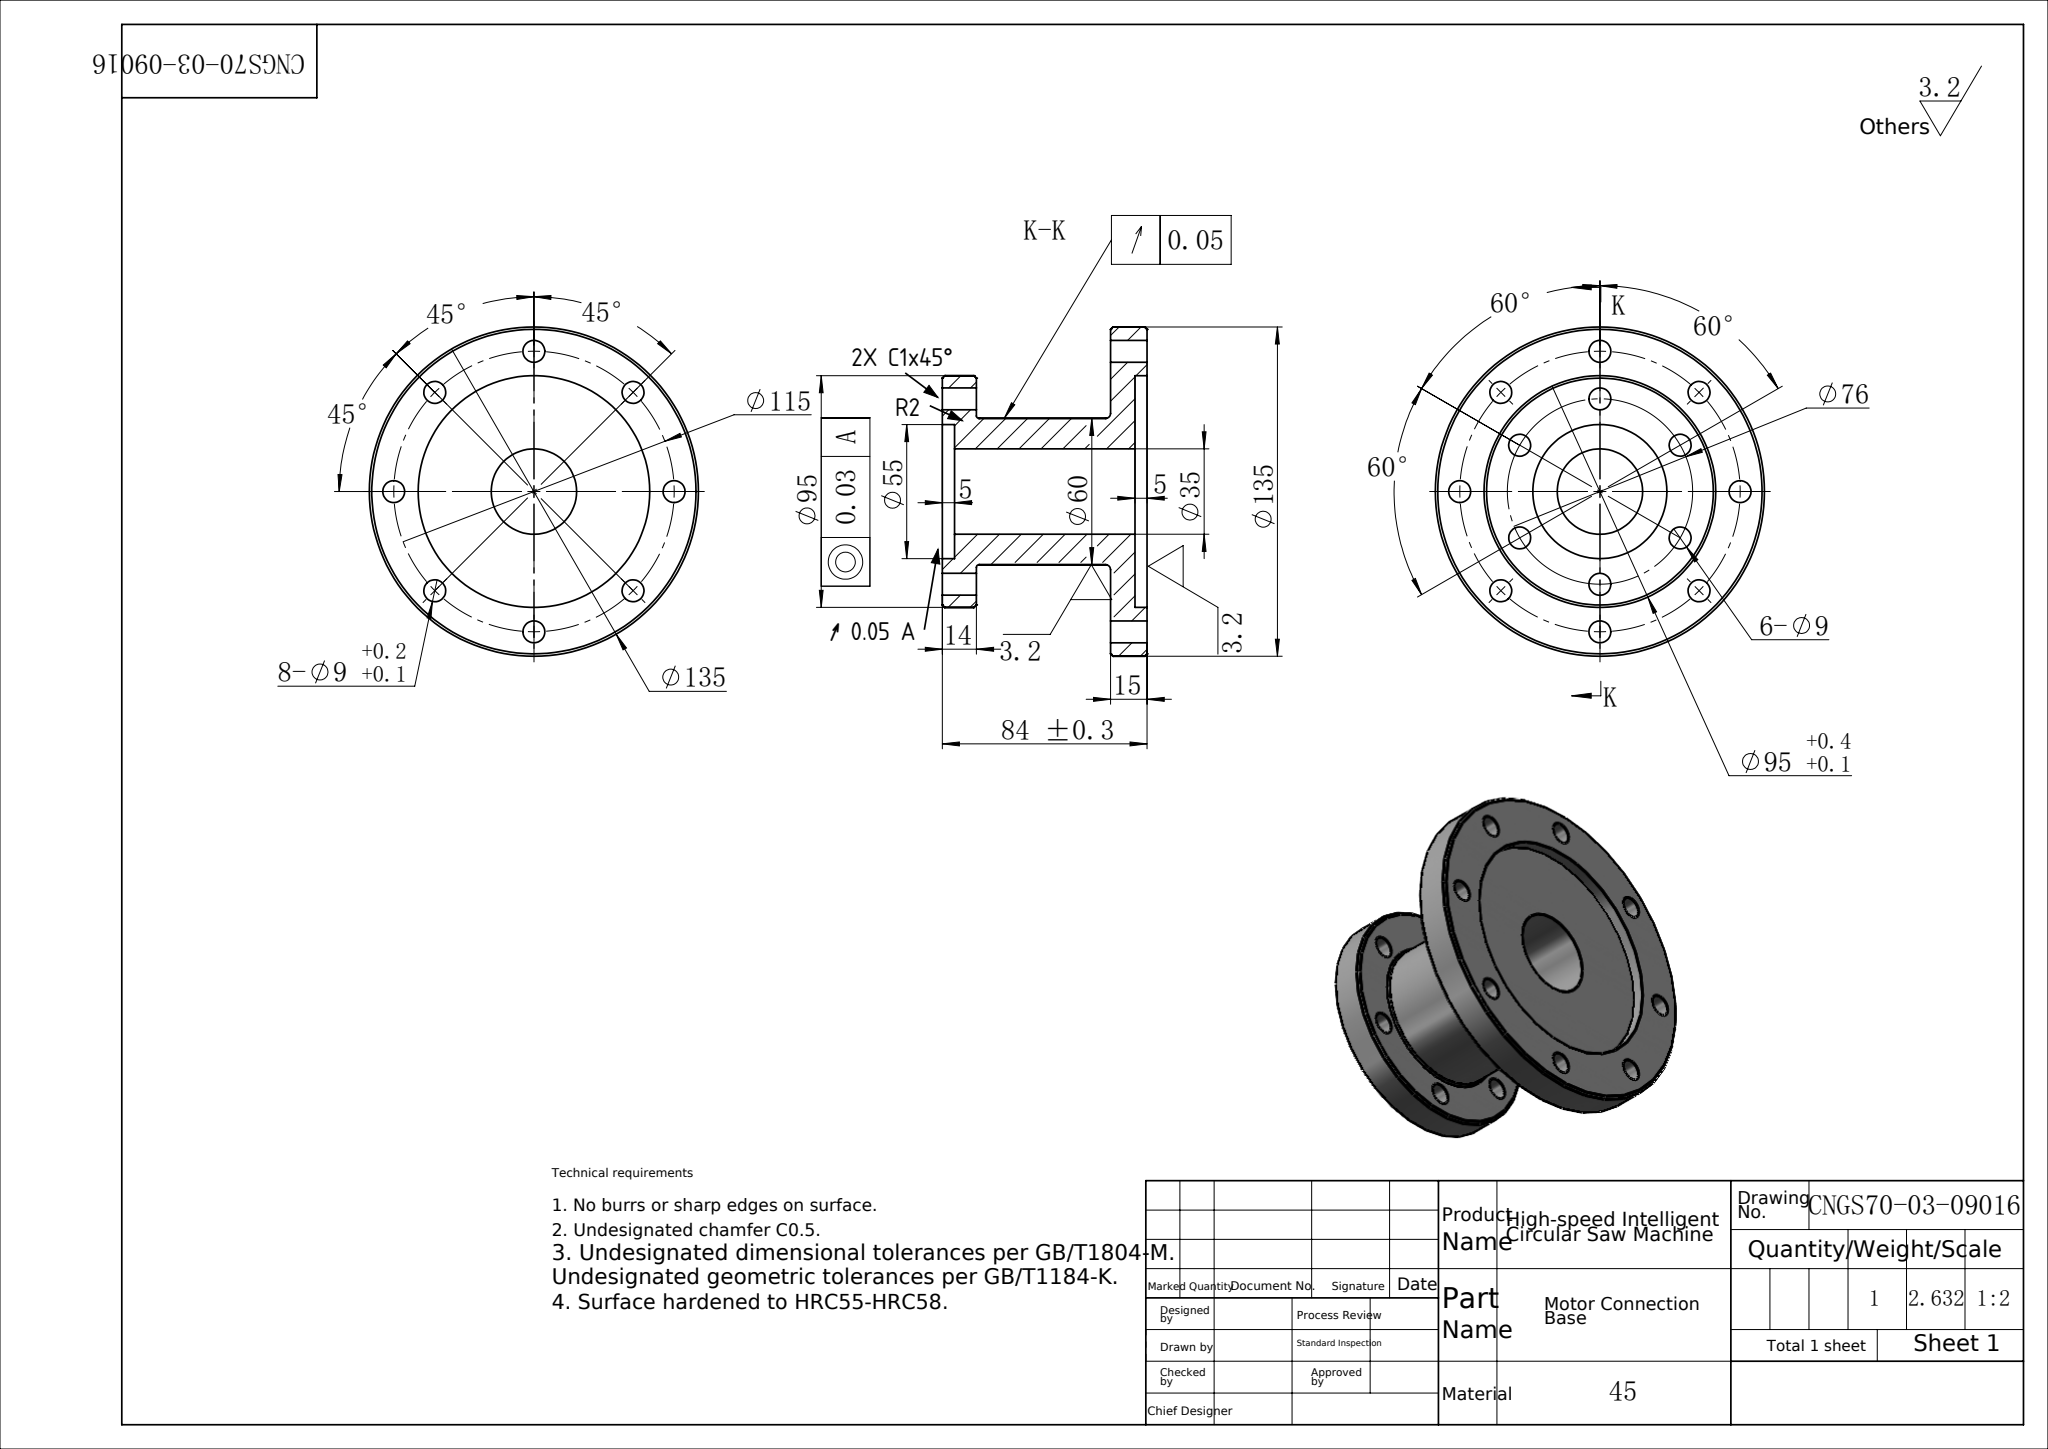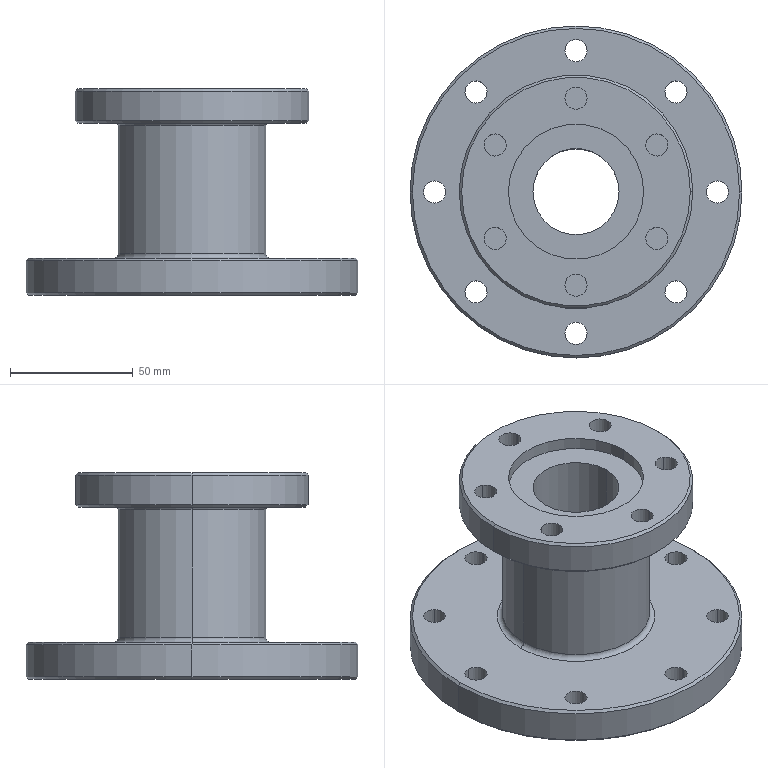Part | SolidWorks | mm | material 45 | 1 solid | 58 faces | box 135 x 135 x 84 mm | volume 337444 mm3 | cylinder 40 | cone 8 | plane 6 | torus 4 | commonest cylinder face diameters 9 x28 95 x4 55 x2 135 x2 60 x2 35 x2
Drawing notes:
K-K: CIRCULAR RUNOUT ↗ 0.05 OF Ø95 FLANGE FACE TO DATUM A | from the solid: Ø95 cyl, axis z at (67.5,67.5), faces at z=0/5 and z=79/84 coaxial with Ø60 hub (L=52) and Ø35 bore (L=74); flange faces are planes normal to z at 0,5,79,84
UNNOTED FILLETS R2 AT HUB-TO-FLANGE TRANSITIONS, R1 ALL OTHERS | from the solid: fillet_radii: [[2.0, 2], [1.0, 2]] - two R2 and two R1 blends on hub/flange junctions in section K-K
C1 x 45° BOTH EDGES OF Ø95 FLANGE (SEE K-K) | from the solid: cones 90° incl, ref dia 95 & 93 (2 ea) at Ø95 flange faces = 1 mm x 45° chamfer
build123d program:
from build123d import *

# Parameters (mm, degrees)
SKETCH1_R                     = 47.5
BOSS_EXTRUDE1_DEPTH           = 14
SIZE_MM_DOWEL_PIN_HOLE1_D     = 9
SIZE_MM_DOWEL_PIN_HOLE1_DEPTH = 14
SKETCH5_R                     = 30
BOSS_EXTRUDE2_DEPTH           = 55
SKETCH6_R                     = 67.5
BOSS_EXTRUDE3_DEPTH           = 15
SKETCH7_R                     = 47.5
CUT_EXTRUDE3_DEPTH            = 5
FILLET1_R                     = 1
FILLET2_R                     = 2
CHAMFER1_SIZE                 = 1
SKETCH10_R                    = 17.5
CUT_EXTRUDE4_DEPTH            = 124.909
SKETCH2_R                     = 31
SKETCH2_R_2                   = 25
BOSS_EXTRUDE4_DEPTH           = 3.5
CUT_EXTRUDE5_START            = -3.5
SKETCH11_R                    = 31
CUT_EXTRUDE5_DEPTH            = 3.5
SKETCH12_R                    = 27.5
CUT_EXTRUDE6_DEPTH            = 5
CIRPATTERN1_COUNT             = 8
CIRPATTERN2_COUNT             = 6


with BuildPart() as part:
    # Sketch1 → Boss-Extrude1 (new body)
    with BuildSketch(Plane.XY):
        Circle(SKETCH1_R)
    extrude(amount=BOSS_EXTRUDE1_DEPTH)

    # Size mm Dowel Pin Hole1
    with Locations(Plane(origin=(0, 0, 0), x_dir=(-1, 0, 0), z_dir=(0, 0, -1))):
        with Locations((0, 38)):
            size_mm_dowel_pin_hole1 = Hole(SIZE_MM_DOWEL_PIN_HOLE1_D / 2, depth=SIZE_MM_DOWEL_PIN_HOLE1_DEPTH)

    # Sketch5 → Boss-Extrude2 (add)
    with BuildSketch(Plane(origin=(0, 0, 0), x_dir=(-1, 0, 0), z_dir=(0, 0, -1))):
        with Locations(Location((0, 0, 0), (0, 0, 180))):
            Circle(SKETCH5_R)
    extrude(amount=BOSS_EXTRUDE2_DEPTH)

    # Sketch6 → Boss-Extrude3 (add)
    with BuildSketch(Plane(origin=(0, 0, -55), x_dir=(-1, 0, 0), z_dir=(0, 0, -1))):
        Circle(SKETCH6_R)
    extrude(amount=BOSS_EXTRUDE3_DEPTH)

    # Sketch7 → Cut-Extrude3 (cut)
    with BuildSketch(Plane(origin=(0, 0, -70), x_dir=(-1, 0, 0), z_dir=(0, 0, -1))):
        with Locations(Location((0, 0, 0), (0, 0, 180))):
            Circle(SKETCH7_R)
    extrude(amount=-CUT_EXTRUDE3_DEPTH, mode=Mode.SUBTRACT)

    # Fillet1
    fillet1_edges = [part.edges().sort_by_distance(p)[0] for p in [
        (-30, 0, 0),
    ]]
    fillet(fillet1_edges, radius=FILLET1_R)

    # Fillet2
    fillet2_edges = [part.edges().sort_by_distance(p)[0] for p in [
        (-30, 0, -55),
    ]]
    fillet(fillet2_edges, radius=FILLET2_R)

    # Chamfer1
    chamfer1_edges = [part.edges().sort_by_distance(p)[0] for p in [
        (67.5, 0, -55),
        (67.5, 0, -70),
        (-47.5, 0, 0),
        (-47.5, 0, 14),
    ]]
    chamfer(chamfer1_edges, length=CHAMFER1_SIZE)

    # Sketch10 → Cut-Extrude4 (cut, through all)
    with BuildSketch(Plane(origin=(0, 0, -65), x_dir=(-1, 0, 0), z_dir=(0, 0, -1))):
        Circle(SKETCH10_R)
    extrude(amount=-CUT_EXTRUDE4_DEPTH, mode=Mode.SUBTRACT)

    # Sketch2 → Boss-Extrude4 (add)
    with BuildSketch(Plane.XY.offset(14)):
        Circle(SKETCH2_R)
        Circle(SKETCH2_R_2, mode=Mode.SUBTRACT)
    extrude(amount=BOSS_EXTRUDE4_DEPTH)

    # Sketch11 → Cut-Extrude5 (cut)
    with BuildSketch(Plane.XY.offset(17.5).offset(CUT_EXTRUDE5_START)):
        Circle(SKETCH11_R)
    extrude(amount=CUT_EXTRUDE5_DEPTH, mode=Mode.SUBTRACT)

    # Sketch12 → Cut-Extrude6 (cut)
    with BuildSketch(Plane.XY.offset(14)):
        Circle(SKETCH12_R)
    extrude(amount=-CUT_EXTRUDE6_DEPTH, mode=Mode.SUBTRACT)

    # Sketch14 → 9.0 _9_ Diameter Hole1 (revolve, cut)
    with BuildSketch(Plane(origin=(0, 57.5, -70), x_dir=(0, 1, 0), z_dir=(1, 0, 0))):
        Polygon((0, 0), (0, 17.704), (4.5, 15), (4.5, 0), align=None)
    f_9_0_9_diameter_hole1 = revolve(axis=Axis((0, 57.5, -76.35), (0, 0, 1)), mode=Mode.SUBTRACT)

    # CirPattern1: 9.0 _9_ Diameter Hole1 ×8 about axis
    cirpattern1_axis = Axis((0, 0, 0), (0, 0, 1))
    for i in range(1, CIRPATTERN1_COUNT):
        add(f_9_0_9_diameter_hole1.rotate(cirpattern1_axis, i * 360 / CIRPATTERN1_COUNT), mode=Mode.SUBTRACT)

    # CirPattern2: Size mm Dowel Pin Hole1 ×6 about axis
    cirpattern2_axis = Axis((0, 0, 0), (0, 0, 1))
    for i in range(1, CIRPATTERN2_COUNT):
        add(size_mm_dowel_pin_hole1.rotate(cirpattern2_axis, i * 360 / CIRPATTERN2_COUNT), mode=Mode.SUBTRACT)


solid = part.part